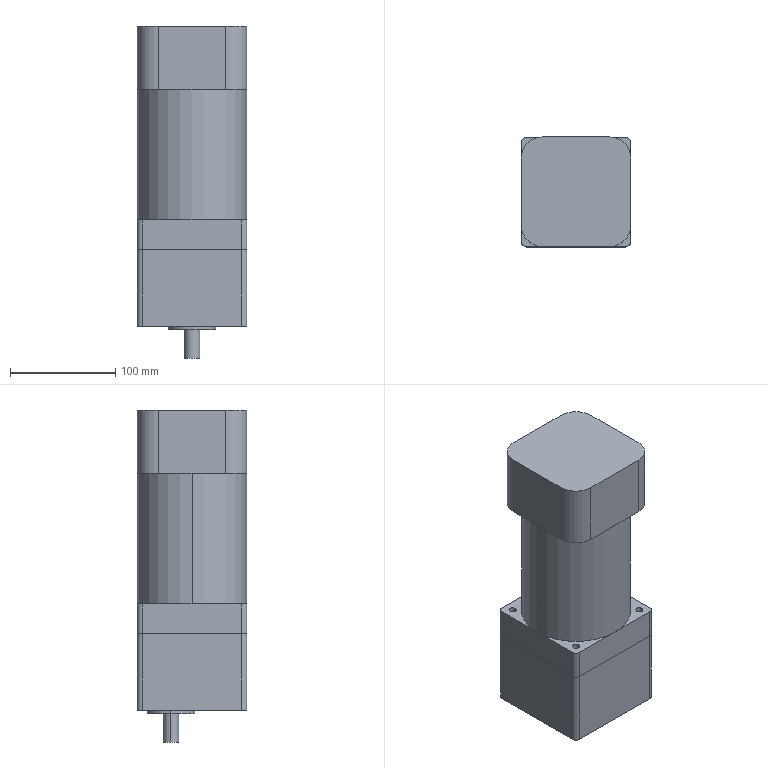Component | SolidWorks | 200WBrakeMotor,-1 | 2 solids | 66 faces | box 104 x 104 x 315 mm | volume 2766388 mm3 | cylinder 38 | plane 28 | commonest cylinder face diameters 6.5 x20 10 x8 40 x4 104 x2 15 x2 45.5 x2
build123d program:
from build123d import *

# Parameters (mm, degrees)
SKETCH1_W                           = 104
SKETCH1_H                           = 104
BOSS_EXTRUDE1_DEPTH                 = 73
SKETCH2_W                           = 104
SKETCH2_H                           = 104
BOSS_EXTRUDE2_DEPTH                 = 212
SKETCH3_W                           = 12
SKETCH3_H                           = 12
CUT_EXTRUDE1_DEPTH                  = 184
SKETCH4_R                           = 73.539
SKETCH4_R_2                         = 52
CUT_EXTRUDE2_DEPTH                  = 184
SKETCH5_W                           = 104
SKETCH5_H                           = 104
BOSS_EXTRUDE3_DEPTH                 = 60
FILLET1_R                           = 20
FILLET2_R                           = 5
FILLET3_R                           = 5
SKETCH6_R                           = 22.75
BOSS_EXTRUDE4_DEPTH                 = 3
SKETCH7_R                           = 7.5
BOSS_EXTRUDE5_DEPTH                 = 27
SKETCH10_W                          = 3.25
SKETCH10_H                          = 131
F_6_5_6_5_DIAMETER_HOLE1_AT_2_COUNT = 2
F_6_5_6_5_DIAMETER_HOLE1_AT_2_PITCH = 60.104
F_6_5_6_5_DIAMETER_HOLE1_AT_3_COUNT = 2
F_6_5_6_5_DIAMETER_HOLE1_AT_3_PITCH = 60.104
F_6_5_6_5_DIAMETER_HOLE1_AT_4_COUNT = 2
F_6_5_6_5_DIAMETER_HOLE1_AT_4_PITCH = 60.104
F_6_5_6_5_DIAMETER_HOLE1_AT_5_COUNT = 2
F_6_5_6_5_DIAMETER_HOLE1_AT_5_PITCH = 60.104
BOSS_EXTRUDE6_START                 = -46
SKETCH11_R                          = 3.25
BOSS_EXTRUDE6_DEPTH                 = 46
BOSS_EXTRUDE9_START                 = -3
SKETCH12_R                          = 22.75
BOSS_EXTRUDE9_DEPTH                 = 3


with BuildPart() as part:
    # Sketch1 → Boss-Extrude1 (new body)
    with BuildSketch(Plane.XY):
        Rectangle(SKETCH1_W, SKETCH1_H)
    extrude(amount=BOSS_EXTRUDE1_DEPTH)

    # Fillet2
    fillet2_edges = [part.edges().sort_by_distance(p)[0] for p in [
        (-52, 52, 36.5),
        (52, 52, 36.5),
        (52, -52, 36.5),
        (-52, -52, 36.5),
    ]]
    fillet(fillet2_edges, radius=FILLET2_R)

    # Sketch6 → Boss-Extrude4 (add)
    with BuildSketch(Plane(origin=(0, 0, 0), x_dir=(-1, 0, 0), z_dir=(0, 0, -1))):
        with Locations(Location((0, -20, 0), (0, 0, 180))):
            Circle(SKETCH6_R)
    extrude(amount=BOSS_EXTRUDE4_DEPTH)

    # Sketch7 → Boss-Extrude5 (add)
    with BuildSketch(Plane(origin=(0, 0, -3), x_dir=(-1, 0, 0), z_dir=(0, 0, -1))):
        with Locations((0, -20)):
            Circle(SKETCH7_R)
    extrude(amount=BOSS_EXTRUDE5_DEPTH)


with BuildPart() as body_2:
    # Sketch2 → Boss-Extrude2 (new body)
    with BuildSketch(Plane.XY.offset(73)):
        Rectangle(SKETCH2_W, SKETCH2_H)
    extrude(amount=BOSS_EXTRUDE2_DEPTH)

    # Sketch3 → Cut-Extrude1 (cut)
    with BuildSketch(Plane.XY.offset(285)):
        with Locations((-46, 46)):
            Rectangle(SKETCH3_W, SKETCH3_H)
        with Locations((46, 46)):
            Rectangle(SKETCH3_W, SKETCH3_H)
        with Locations((-46, -46)):
            Rectangle(SKETCH3_W, SKETCH3_H)
        with Locations((46, -46)):
            Rectangle(SKETCH3_W, SKETCH3_H)
    extrude(amount=-CUT_EXTRUDE1_DEPTH, mode=Mode.SUBTRACT)

    # Sketch4 → Cut-Extrude2 (cut)
    with BuildSketch(Plane.XY.offset(285)):
        Circle(SKETCH4_R)
        Circle(SKETCH4_R_2, mode=Mode.SUBTRACT)
    extrude(amount=-CUT_EXTRUDE2_DEPTH, mode=Mode.SUBTRACT)

    # Sketch5 → Boss-Extrude3 (add)
    with BuildSketch(Plane.XY.offset(285)):
        Rectangle(SKETCH5_W, SKETCH5_H)
    extrude(amount=-BOSS_EXTRUDE3_DEPTH)

    # Fillet1
    fillet1_edges = [body_2.edges().sort_by_distance(p)[0] for p in [
        (-52, -52, 255),
        (-52, 52, 255),
        (52, 52, 255),
        (52, -52, 255),
    ]]
    fillet(fillet1_edges, radius=FILLET1_R)

    # Fillet3
    fillet3_edges = [body_2.edges().sort_by_distance(p)[0] for p in [
        (-52, 52, 87),
        (52, 52, 87),
        (52, -52, 87),
        (-52, -52, 87),
    ]]
    fillet(fillet3_edges, radius=FILLET3_R)


with BuildPart() as f_6_5_6_5_diameter_hole1_tool:
    # Sketch10 → 6.5 _6.5_ Diameter Hole1 (revolve)
    with BuildSketch(Plane(origin=(0, 0, 101), x_dir=(0, -1, 0), z_dir=(1, 0, 0))):
        with Locations((1.625, 65.5)):
            Rectangle(SKETCH10_W, SKETCH10_H)
    f_6_5_6_5_diameter_hole1 = revolve(axis=Axis((0, 0, 107.35), (0, 0, -1)))


with BuildPart() as part_1:
    add(part.part)

    # 6.5 _6.5_ Diameter Hole1: cut by f_6_5_6_5_diameter_hole1_tool
    add(f_6_5_6_5_diameter_hole1_tool.part, mode=Mode.SUBTRACT)


with BuildPart() as body_2_1:
    add(body_2.part)

    # 6.5 _6.5_ Diameter Hole1: cut by f_6_5_6_5_diameter_hole1_tool
    add(f_6_5_6_5_diameter_hole1_tool.part, mode=Mode.SUBTRACT)


with BuildPart() as f_6_5_6_5_diameter_hole1_at_2_tool:
    # 6.5 _6.5_ Diameter Hole1 at 2: 6.5 _6.5_ Diameter Hole1 ×2
    with Locations(*[Vector(-0.7071, 0.7071, 0) * (i * F_6_5_6_5_DIAMETER_HOLE1_AT_2_PITCH) for i in range(1, F_6_5_6_5_DIAMETER_HOLE1_AT_2_COUNT)]):
        add(f_6_5_6_5_diameter_hole1)


with BuildPart() as part_2:
    add(part_1.part)

    # 6.5 _6.5_ Diameter Hole1 at 2: cut by f_6_5_6_5_diameter_hole1_at_2_tool
    add(f_6_5_6_5_diameter_hole1_at_2_tool.part, mode=Mode.SUBTRACT)


with BuildPart() as body_2_2:
    add(body_2_1.part)

    # 6.5 _6.5_ Diameter Hole1 at 2: cut by f_6_5_6_5_diameter_hole1_at_2_tool
    add(f_6_5_6_5_diameter_hole1_at_2_tool.part, mode=Mode.SUBTRACT)


with BuildPart() as f_6_5_6_5_diameter_hole1_at_3_tool:
    # 6.5 _6.5_ Diameter Hole1 at 3: 6.5 _6.5_ Diameter Hole1 ×2
    with Locations(*[Vector(0.7071, -0.7071, 0) * (i * F_6_5_6_5_DIAMETER_HOLE1_AT_3_PITCH) for i in range(1, F_6_5_6_5_DIAMETER_HOLE1_AT_3_COUNT)]):
        add(f_6_5_6_5_diameter_hole1)


with BuildPart() as part_3:
    add(part_2.part)

    # 6.5 _6.5_ Diameter Hole1 at 3: cut by f_6_5_6_5_diameter_hole1_at_3_tool
    add(f_6_5_6_5_diameter_hole1_at_3_tool.part, mode=Mode.SUBTRACT)


with BuildPart() as body_2_3:
    add(body_2_2.part)

    # 6.5 _6.5_ Diameter Hole1 at 3: cut by f_6_5_6_5_diameter_hole1_at_3_tool
    add(f_6_5_6_5_diameter_hole1_at_3_tool.part, mode=Mode.SUBTRACT)


with BuildPart() as f_6_5_6_5_diameter_hole1_at_4_tool:
    # 6.5 _6.5_ Diameter Hole1 at 4: 6.5 _6.5_ Diameter Hole1 ×2
    with Locations(*[Vector(0.7071, 0.7071, 0) * (i * F_6_5_6_5_DIAMETER_HOLE1_AT_4_PITCH) for i in range(1, F_6_5_6_5_DIAMETER_HOLE1_AT_4_COUNT)]):
        add(f_6_5_6_5_diameter_hole1)


with BuildPart() as part_4:
    add(part_3.part)

    # 6.5 _6.5_ Diameter Hole1 at 4: cut by f_6_5_6_5_diameter_hole1_at_4_tool
    add(f_6_5_6_5_diameter_hole1_at_4_tool.part, mode=Mode.SUBTRACT)


with BuildPart() as body_2_4:
    add(body_2_3.part)

    # 6.5 _6.5_ Diameter Hole1 at 4: cut by f_6_5_6_5_diameter_hole1_at_4_tool
    add(f_6_5_6_5_diameter_hole1_at_4_tool.part, mode=Mode.SUBTRACT)


with BuildPart() as f_6_5_6_5_diameter_hole1_at_5_tool:
    # 6.5 _6.5_ Diameter Hole1 at 5: 6.5 _6.5_ Diameter Hole1 ×2
    with Locations(*[Vector(-0.7071, -0.7071, 0) * (i * F_6_5_6_5_DIAMETER_HOLE1_AT_5_PITCH) for i in range(1, F_6_5_6_5_DIAMETER_HOLE1_AT_5_COUNT)]):
        add(f_6_5_6_5_diameter_hole1)


with BuildPart() as part_5:
    add(part_4.part)

    # 6.5 _6.5_ Diameter Hole1 at 5: cut by f_6_5_6_5_diameter_hole1_at_5_tool
    add(f_6_5_6_5_diameter_hole1_at_5_tool.part, mode=Mode.SUBTRACT)

    # Sketch11 → Boss-Extrude6 (add)
    with BuildSketch(Plane(origin=(0, 0, 0), x_dir=(-1, 0, 0), z_dir=(0, 0, -1)).offset(BOSS_EXTRUDE6_START)):
        with Locations(Location((0, 0, 0), (0, 0, 180))):
            Circle(SKETCH11_R)
    extrude(amount=BOSS_EXTRUDE6_DEPTH)

    # Sketch12 → Boss-Extrude9 (add)
    with BuildSketch(Plane(origin=(0, 0, -3), x_dir=(-1, 0, 0), z_dir=(0, 0, -1)).offset(BOSS_EXTRUDE9_START)):
        with Locations(Location((0, -20, 0), (0, 0, 180))):
            Circle(SKETCH12_R)
    extrude(amount=BOSS_EXTRUDE9_DEPTH)


with BuildPart() as body_2_5:
    add(body_2_4.part)

    # 6.5 _6.5_ Diameter Hole1 at 5: cut by f_6_5_6_5_diameter_hole1_at_5_tool
    add(f_6_5_6_5_diameter_hole1_at_5_tool.part, mode=Mode.SUBTRACT)


solid = Compound([part_5.part, body_2_5.part])

# Placed as in the assembly
solid = solid.moved(Location((-25.633, -394.591, 61), (0, 0, 180)))